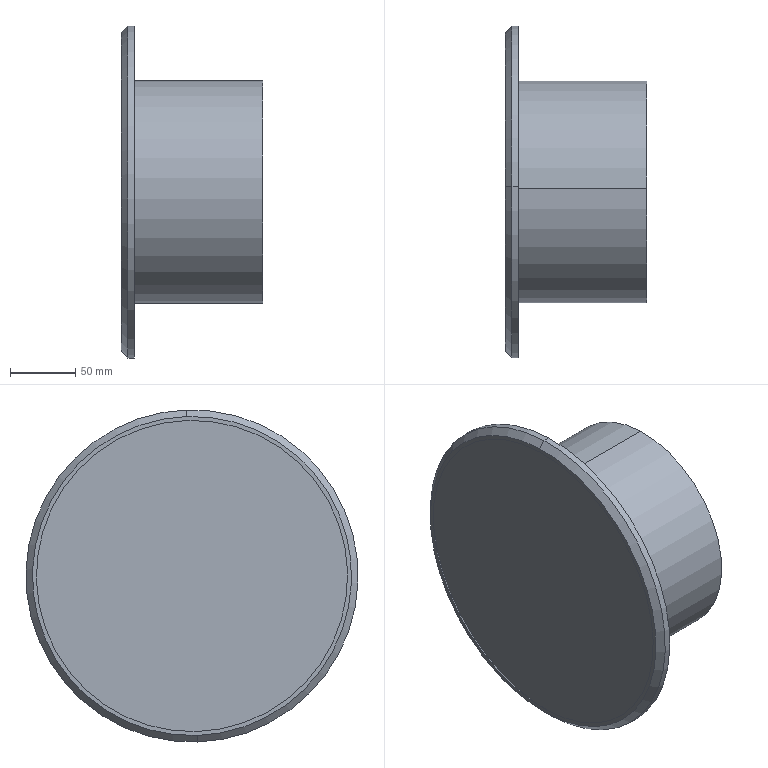Component | SolidWorks | Liner-1 | 1 solid | 15 faces | box 108 x 254 x 254 mm | volume 805465 mm3 | cylinder 6 | plane 5 | cone 4 | commonest cylinder face diameters 254 x2 170 x2 150 x2
build123d program:
from build123d import *

# Parameters (mm, degrees)
CHAMFER2_SIZE = 5


with BuildPart() as part:
    # Sketch1 → Revolve1 (revolve)
    with BuildSketch(Plane.XY, mode=Mode.PRIVATE) as revolve1_sk:
        Polygon((108, 75), (108, 85), (10, 85), (10, 127), (0, 127), (0, 119), (4, 123), (4, 0), (10, 0), (10, 75), align=None)
    revolve(revolve1_sk.sketch.rotate(Axis((0, 0, 0), (1, 0, 0)), 90), axis=Axis((0, 0, 0), (1, 0, 0)))

    # Chamfer2
    chamfer2_edges = [part.edges().sort_by_distance(p)[0] for p in [
        (0, 0, -127),
    ]]
    chamfer(chamfer2_edges, length=CHAMFER2_SIZE)


solid = part.part

# Placed as in the assembly
solid = solid.moved(Location((-257.5, 0, 0), (0, 0, 0)))
STEP:
#1=COLOUR_RGB('',0.7922,0.8196,0.9333);
#2=FILL_AREA_STYLE_COLOUR('',#1);
#3=FILL_AREA_STYLE('',(#2));
#4=SURFACE_STYLE_FILL_AREA(#3);
#5=SURFACE_SIDE_STYLE('',(#4));
#6=SURFACE_STYLE_USAGE(.BOTH.,#5);
#7=PRESENTATION_STYLE_ASSIGNMENT((#6));
#8=CARTESIAN_POINT('',(-10.138,0.1561,4.801));
#9=VERTEX_POINT('',#8);
#10=CARTESIAN_POINT('',(-10.138,-0.1561,-4.801));
#11=VERTEX_POINT('',#10);
#12=CARTESIAN_POINT('',(-10.138,-0.,0.));
#13=DIRECTION('',(-1.,-0.,0.));
#14=DIRECTION('',(-0.,-0.0325,-0.9995));
#15=AXIS2_PLACEMENT_3D('',#12,#13,#14);
#16=CIRCLE('',#15,4.803);
#17=EDGE_CURVE('',#9,#11,#16,.T.);
#18=ORIENTED_EDGE('',*,*,#17,.F.);
#19=CARTESIAN_POINT('',(-9.941,0.1625,4.997));
#20=VERTEX_POINT('',#19);
#21=CARTESIAN_POINT('',(-10.138,0.1561,4.801));
#22=DIRECTION('',(0.7071,0.02298,0.7067));
#23=VECTOR('',#22,39.37);
#24=LINE('',#21,#23);
#25=EDGE_CURVE('',#9,#20,#24,.T.);
#26=ORIENTED_EDGE('',*,*,#25,.T.);
#27=CARTESIAN_POINT('',(-9.941,-0.1625,-4.997));
#28=VERTEX_POINT('',#27);
#29=CARTESIAN_POINT('',(-9.941,-0.,0.));
#30=DIRECTION('',(1.,0.,-0.));
#31=DIRECTION('',(-0.,-0.0325,-0.9995));
#32=AXIS2_PLACEMENT_3D('',#29,#30,#31);
#33=CIRCLE('',#32,5.);
#34=EDGE_CURVE('',#28,#20,#33,.T.);
#35=ORIENTED_EDGE('',*,*,#34,.F.);
#36=CARTESIAN_POINT('',(-10.138,-0.1561,-4.801));
#37=DIRECTION('',(0.7071,-0.02298,-0.7067));
#38=VECTOR('',#37,39.37);
#39=LINE('',#36,#38);
#40=EDGE_CURVE('',#11,#28,#39,.T.);
#41=ORIENTED_EDGE('',*,*,#40,.F.);
#42=EDGE_LOOP('',(#18,#26,#35,#41));
#43=FACE_OUTER_BOUND('',#42,.T.);
#44=CARTESIAN_POINT('',(-10.138,-0.,0.));
#45=DIRECTION('',(1.,0.,-0.));
#46=DIRECTION('',(-0.,-0.0325,-0.9995));
#47=AXIS2_PLACEMENT_3D('',#44,#45,#46);
#48=CONICAL_SURFACE('',#47,4.803,0.7854);
#49=ADVANCED_FACE('',(#43),#48,.T.);
#50=CARTESIAN_POINT('',(-10.138,-0.1523,-4.683));
#51=VERTEX_POINT('',#50);
#52=CARTESIAN_POINT('',(-10.138,0.1523,4.683));
#53=VERTEX_POINT('',#52);
#54=CARTESIAN_POINT('',(-10.138,-0.,0.));
#55=DIRECTION('',(-1.,-0.,0.));
#56=DIRECTION('',(0.,0.0325,0.9995));
#57=AXIS2_PLACEMENT_3D('',#54,#55,#56);
#58=CIRCLE('',#57,4.685);
#59=EDGE_CURVE('',#51,#53,#58,.T.);
#60=ORIENTED_EDGE('',*,*,#59,.T.);
#61=CARTESIAN_POINT('',(-9.98,0.1574,4.84));
#62=VERTEX_POINT('',#61);
#63=CARTESIAN_POINT('',(-10.138,0.1523,4.683));
#64=DIRECTION('',(0.7071,0.02298,0.7067));
#65=VECTOR('',#64,39.37);
#66=LINE('',#63,#65);
#67=EDGE_CURVE('',#53,#62,#66,.T.);
#68=ORIENTED_EDGE('',*,*,#67,.T.);
#69=CARTESIAN_POINT('',(-9.98,-0.1574,-4.84));
#70=VERTEX_POINT('',#69);
#71=CARTESIAN_POINT('',(-9.98,-0.,0.));
#72=DIRECTION('',(-1.,-0.,0.));
#73=DIRECTION('',(0.,0.0325,0.9995));
#74=AXIS2_PLACEMENT_3D('',#71,#72,#73);
#75=CIRCLE('',#74,4.843);
#76=EDGE_CURVE('',#70,#62,#75,.T.);
#77=ORIENTED_EDGE('',*,*,#76,.F.);
#78=CARTESIAN_POINT('',(-10.138,-0.1523,-4.683));
#79=DIRECTION('',(0.7071,-0.02298,-0.7067));
#80=VECTOR('',#79,39.37);
#81=LINE('',#78,#80);
#82=EDGE_CURVE('',#51,#70,#81,.T.);
#83=ORIENTED_EDGE('',*,*,#82,.F.);
#84=EDGE_LOOP('',(#60,#68,#77,#83));
#85=FACE_OUTER_BOUND('',#84,.T.);
#86=CARTESIAN_POINT('',(-10.138,-0.,0.));
#87=DIRECTION('',(1.,0.,-0.));
#88=DIRECTION('',(-0.,-0.0325,-0.9995));
#89=AXIS2_PLACEMENT_3D('',#86,#87,#88);
#90=CONICAL_SURFACE('',#89,4.685,0.7854);
#91=ADVANCED_FACE('',(#85),#90,.F.);
#92=CARTESIAN_POINT('',(-9.744,0.1625,4.997));
#93=VERTEX_POINT('',#92);
#94=CARTESIAN_POINT('',(-9.744,-0.1625,-4.997));
#95=VERTEX_POINT('',#94);
#96=CARTESIAN_POINT('',(-9.744,-0.,0.));
#97=DIRECTION('',(-1.,-0.,0.));
#98=DIRECTION('',(0.,0.0325,0.9995));
#99=AXIS2_PLACEMENT_3D('',#96,#97,#98);
#100=CIRCLE('',#99,5.);
#101=EDGE_CURVE('',#93,#95,#100,.T.);
#102=ORIENTED_EDGE('',*,*,#101,.T.);
#103=CARTESIAN_POINT('',(-10.138,-0.1625,-4.997));
#104=DIRECTION('',(-1.,-0.,0.));
#105=VECTOR('',#104,39.37);
#106=LINE('',#103,#105);
#107=EDGE_CURVE('',#95,#28,#106,.T.);
#108=ORIENTED_EDGE('',*,*,#107,.T.);
#109=ORIENTED_EDGE('',*,*,#34,.T.);
#110=CARTESIAN_POINT('',(-10.138,0.1625,4.997));
#111=DIRECTION('',(-1.,-0.,0.));
#112=VECTOR('',#111,39.37);
#113=LINE('',#110,#112);
#114=EDGE_CURVE('',#93,#20,#113,.T.);
#115=ORIENTED_EDGE('',*,*,#114,.F.);
#116=EDGE_LOOP('',(#102,#108,#109,#115));
#117=FACE_OUTER_BOUND('',#116,.T.);
#118=CARTESIAN_POINT('',(-10.138,-0.,0.));
#119=DIRECTION('',(-1.,-0.,0.));
#120=DIRECTION('',(0.,0.0325,0.9995));
#121=AXIS2_PLACEMENT_3D('',#118,#119,#120);
#122=CYLINDRICAL_SURFACE('',#121,5.);
#123=ADVANCED_FACE('',(#117),#122,.T.);
#124=CARTESIAN_POINT('',(-5.886,0.1088,3.345));
#125=VERTEX_POINT('',#124);
#126=CARTESIAN_POINT('',(-5.886,-0.1088,-3.345));
#127=VERTEX_POINT('',#126);
#128=CARTESIAN_POINT('',(-5.886,-0.,0.));
#129=DIRECTION('',(-1.,-0.,0.));
#130=DIRECTION('',(0.,0.0325,0.9995));
#131=AXIS2_PLACEMENT_3D('',#128,#129,#130);
#132=CIRCLE('',#131,3.346);
#133=EDGE_CURVE('',#125,#127,#132,.T.);
#134=ORIENTED_EDGE('',*,*,#133,.T.);
#135=CARTESIAN_POINT('',(-9.744,-0.1088,-3.345));
#136=VERTEX_POINT('',#135);
#137=CARTESIAN_POINT('',(-10.138,-0.1088,-3.345));
#138=DIRECTION('',(-1.,-0.,0.));
#139=VECTOR('',#138,39.37);
#140=LINE('',#137,#139);
#141=EDGE_CURVE('',#127,#136,#140,.T.);
#142=ORIENTED_EDGE('',*,*,#141,.T.);
#143=CARTESIAN_POINT('',(-9.744,0.1088,3.345));
#144=VERTEX_POINT('',#143);
#145=CARTESIAN_POINT('',(-9.744,-0.,0.));
#146=DIRECTION('',(-1.,-0.,0.));
#147=DIRECTION('',(0.,0.0325,0.9995));
#148=AXIS2_PLACEMENT_3D('',#145,#146,#147);
#149=CIRCLE('',#148,3.346);
#150=EDGE_CURVE('',#144,#136,#149,.T.);
#151=ORIENTED_EDGE('',*,*,#150,.F.);
#152=CARTESIAN_POINT('',(-10.138,0.1088,3.345));
#153=DIRECTION('',(-1.,-0.,0.));
#154=VECTOR('',#153,39.37);
#155=LINE('',#152,#154);
#156=EDGE_CURVE('',#125,#144,#155,.T.);
#157=ORIENTED_EDGE('',*,*,#156,.F.);
#158=EDGE_LOOP('',(#134,#142,#151,#157));
#159=FACE_OUTER_BOUND('',#158,.T.);
#160=CARTESIAN_POINT('',(-10.138,-0.,0.));
#161=DIRECTION('',(-1.,-0.,0.));
#162=DIRECTION('',(0.,0.0325,0.9995));
#163=AXIS2_PLACEMENT_3D('',#160,#161,#162);
#164=CYLINDRICAL_SURFACE('',#163,3.346);
#165=ADVANCED_FACE('',(#159),#164,.T.);
#166=CARTESIAN_POINT('',(-5.886,-0.09596,-2.951));
#167=VERTEX_POINT('',#166);
#168=CARTESIAN_POINT('',(-5.886,0.09596,2.951));
#169=VERTEX_POINT('',#168);
#170=CARTESIAN_POINT('',(-5.886,-0.,0.));
#171=DIRECTION('',(-1.,-0.,0.));
#172=DIRECTION('',(0.,0.0325,0.9995));
#173=AXIS2_PLACEMENT_3D('',#170,#171,#172);
#174=CIRCLE('',#173,2.953);
#175=EDGE_CURVE('',#167,#169,#174,.T.);
#176=ORIENTED_EDGE('',*,*,#175,.F.);
#177=CARTESIAN_POINT('',(-9.744,-0.09596,-2.951));
#178=VERTEX_POINT('',#177);
#179=CARTESIAN_POINT('',(-10.138,-0.09596,-2.951));
#180=DIRECTION('',(-1.,-0.,0.));
#181=VECTOR('',#180,39.37);
#182=LINE('',#179,#181);
#183=EDGE_CURVE('',#167,#178,#182,.T.);
#184=ORIENTED_EDGE('',*,*,#183,.T.);
#185=CARTESIAN_POINT('',(-9.744,0.09596,2.951));
#186=VERTEX_POINT('',#185);
#187=CARTESIAN_POINT('',(-9.744,-0.,0.));
#188=DIRECTION('',(-1.,-0.,0.));
#189=DIRECTION('',(0.,0.0325,0.9995));
#190=AXIS2_PLACEMENT_3D('',#187,#188,#189);
#191=CIRCLE('',#190,2.953);
#192=EDGE_CURVE('',#178,#186,#191,.T.);
#193=ORIENTED_EDGE('',*,*,#192,.T.);
#194=CARTESIAN_POINT('',(-10.138,0.09596,2.951));
#195=DIRECTION('',(-1.,-0.,0.));
#196=VECTOR('',#195,39.37);
#197=LINE('',#194,#196);
#198=EDGE_CURVE('',#169,#186,#197,.T.);
#199=ORIENTED_EDGE('',*,*,#198,.F.);
#200=EDGE_LOOP('',(#176,#184,#193,#199));
#201=FACE_OUTER_BOUND('',#200,.T.);
#202=CARTESIAN_POINT('',(-10.138,-0.,0.));
#203=DIRECTION('',(-1.,-0.,0.));
#204=DIRECTION('',(0.,0.0325,0.9995));
#205=AXIS2_PLACEMENT_3D('',#202,#203,#204);
#206=CYLINDRICAL_SURFACE('',#205,2.953);
#207=ADVANCED_FACE('',(#201),#206,.F.);
#208=ORIENTED_EDGE('',*,*,#183,.F.);
#209=CARTESIAN_POINT('',(-5.886,-0.,0.));
#210=DIRECTION('',(-1.,-0.,0.));
#211=DIRECTION('',(0.,0.0325,0.9995));
#212=AXIS2_PLACEMENT_3D('',#209,#210,#211);
#213=CIRCLE('',#212,2.953);
#214=EDGE_CURVE('',#169,#167,#213,.T.);
#215=ORIENTED_EDGE('',*,*,#214,.F.);
#216=ORIENTED_EDGE('',*,*,#198,.T.);
#217=CARTESIAN_POINT('',(-9.744,-0.,0.));
#218=DIRECTION('',(-1.,-0.,0.));
#219=DIRECTION('',(0.,0.0325,0.9995));
#220=AXIS2_PLACEMENT_3D('',#217,#218,#219);
#221=CIRCLE('',#220,2.953);
#222=EDGE_CURVE('',#186,#178,#221,.T.);
#223=ORIENTED_EDGE('',*,*,#222,.T.);
#224=EDGE_LOOP('',(#208,#215,#216,#223));
#225=FACE_OUTER_BOUND('',#224,.T.);
#226=CARTESIAN_POINT('',(-10.138,-0.,0.));
#227=DIRECTION('',(-1.,-0.,0.));
#228=DIRECTION('',(0.,0.0325,0.9995));
#229=AXIS2_PLACEMENT_3D('',#226,#227,#228);
#230=CYLINDRICAL_SURFACE('',#229,2.953);
#231=ADVANCED_FACE('',(#225),#230,.F.);
#232=ORIENTED_EDGE('',*,*,#133,.F.);
#233=CARTESIAN_POINT('',(-5.886,-0.,0.));
#234=DIRECTION('',(-1.,-0.,0.));
#235=DIRECTION('',(0.,0.0325,0.9995));
#236=AXIS2_PLACEMENT_3D('',#233,#234,#235);
#237=CIRCLE('',#236,3.346);
#238=EDGE_CURVE('',#127,#125,#237,.T.);
#239=ORIENTED_EDGE('',*,*,#238,.F.);
#240=EDGE_LOOP('',(#232,#239));
#241=FACE_OUTER_BOUND('',#240,.T.);
#242=ORIENTED_EDGE('',*,*,#214,.T.);
#243=ORIENTED_EDGE('',*,*,#175,.T.);
#244=EDGE_LOOP('',(#242,#243));
#245=FACE_BOUND('',#244,.T.);
#246=CARTESIAN_POINT('',(-5.886,2.951,-0.09596));
#247=DIRECTION('',(-1.,-0.,0.));
#248=DIRECTION('',(0.,0.0325,0.9995));
#249=AXIS2_PLACEMENT_3D('',#246,#247,#248);
#250=PLANE('',#249);
#251=ADVANCED_FACE('',(#241,#245),#250,.F.);
#252=ORIENTED_EDGE('',*,*,#141,.F.);
#253=ORIENTED_EDGE('',*,*,#238,.T.);
#254=ORIENTED_EDGE('',*,*,#156,.T.);
#255=CARTESIAN_POINT('',(-9.744,-0.,0.));
#256=DIRECTION('',(-1.,-0.,0.));
#257=DIRECTION('',(0.,0.0325,0.9995));
#258=AXIS2_PLACEMENT_3D('',#255,#256,#257);
#259=CIRCLE('',#258,3.346);
#260=EDGE_CURVE('',#136,#144,#259,.T.);
#261=ORIENTED_EDGE('',*,*,#260,.F.);
#262=EDGE_LOOP('',(#252,#253,#254,#261));
#263=FACE_OUTER_BOUND('',#262,.T.);
#264=CARTESIAN_POINT('',(-10.138,-0.,0.));
#265=DIRECTION('',(-1.,-0.,0.));
#266=DIRECTION('',(0.,0.0325,0.9995));
#267=AXIS2_PLACEMENT_3D('',#264,#265,#266);
#268=CYLINDRICAL_SURFACE('',#267,3.346);
#269=ADVANCED_FACE('',(#263),#268,.T.);
#270=ORIENTED_EDGE('',*,*,#101,.F.);
#271=CARTESIAN_POINT('',(-9.744,-0.,0.));
#272=DIRECTION('',(-1.,-0.,0.));
#273=DIRECTION('',(0.,0.0325,0.9995));
#274=AXIS2_PLACEMENT_3D('',#271,#272,#273);
#275=CIRCLE('',#274,5.);
#276=EDGE_CURVE('',#95,#93,#275,.T.);
#277=ORIENTED_EDGE('',*,*,#276,.F.);
#278=EDGE_LOOP('',(#270,#277));
#279=FACE_OUTER_BOUND('',#278,.T.);
#280=ORIENTED_EDGE('',*,*,#150,.T.);
#281=ORIENTED_EDGE('',*,*,#260,.T.);
#282=EDGE_LOOP('',(#280,#281));
#283=FACE_BOUND('',#282,.T.);
#284=CARTESIAN_POINT('',(-9.744,3.345,-0.1088));
#285=DIRECTION('',(-1.,-0.,0.));
#286=DIRECTION('',(0.,0.0325,0.9995));
#287=AXIS2_PLACEMENT_3D('',#284,#285,#286);
#288=PLANE('',#287);
#289=ADVANCED_FACE('',(#279,#283),#288,.F.);
#290=ORIENTED_EDGE('',*,*,#107,.F.);
#291=ORIENTED_EDGE('',*,*,#276,.T.);
#292=ORIENTED_EDGE('',*,*,#114,.T.);
#293=CARTESIAN_POINT('',(-9.941,-0.,0.));
#294=DIRECTION('',(1.,0.,-0.));
#295=DIRECTION('',(-0.,-0.0325,-0.9995));
#296=AXIS2_PLACEMENT_3D('',#293,#294,#295);
#297=CIRCLE('',#296,5.);
#298=EDGE_CURVE('',#20,#28,#297,.T.);
#299=ORIENTED_EDGE('',*,*,#298,.T.);
#300=EDGE_LOOP('',(#290,#291,#292,#299));
#301=FACE_OUTER_BOUND('',#300,.T.);
#302=CARTESIAN_POINT('',(-10.138,-0.,0.));
#303=DIRECTION('',(-1.,-0.,0.));
#304=DIRECTION('',(0.,0.0325,0.9995));
#305=AXIS2_PLACEMENT_3D('',#302,#303,#304);
#306=CYLINDRICAL_SURFACE('',#305,5.);
#307=ADVANCED_FACE('',(#301),#306,.T.);
#308=CARTESIAN_POINT('',(-10.138,-0.,0.));
#309=DIRECTION('',(-1.,-0.,0.));
#310=DIRECTION('',(-0.,-0.0325,-0.9995));
#311=AXIS2_PLACEMENT_3D('',#308,#309,#310);
#312=CIRCLE('',#311,4.803);
#313=EDGE_CURVE('',#11,#9,#312,.T.);
#314=ORIENTED_EDGE('',*,*,#313,.T.);
#315=ORIENTED_EDGE('',*,*,#17,.T.);
#316=EDGE_LOOP('',(#314,#315));
#317=FACE_OUTER_BOUND('',#316,.T.);
#318=ORIENTED_EDGE('',*,*,#59,.F.);
#319=CARTESIAN_POINT('',(-10.138,-0.,0.));
#320=DIRECTION('',(-1.,-0.,0.));
#321=DIRECTION('',(0.,0.0325,0.9995));
#322=AXIS2_PLACEMENT_3D('',#319,#320,#321);
#323=CIRCLE('',#322,4.685);
#324=EDGE_CURVE('',#53,#51,#323,.T.);
#325=ORIENTED_EDGE('',*,*,#324,.F.);
#326=EDGE_LOOP('',(#318,#325));
#327=FACE_BOUND('',#326,.T.);
#328=CARTESIAN_POINT('',(-10.138,4.997,-0.1625));
#329=DIRECTION('',(1.,0.,-0.));
#330=DIRECTION('',(-0.,-0.0325,-0.9995));
#331=AXIS2_PLACEMENT_3D('',#328,#329,#330);
#332=PLANE('',#331);
#333=ADVANCED_FACE('',(#317,#327),#332,.F.);
#334=ORIENTED_EDGE('',*,*,#67,.F.);
#335=ORIENTED_EDGE('',*,*,#324,.T.);
#336=ORIENTED_EDGE('',*,*,#82,.T.);
#337=CARTESIAN_POINT('',(-9.98,-0.,0.));
#338=DIRECTION('',(-1.,-0.,0.));
#339=DIRECTION('',(0.,0.0325,0.9995));
#340=AXIS2_PLACEMENT_3D('',#337,#338,#339);
#341=CIRCLE('',#340,4.843);
#342=EDGE_CURVE('',#62,#70,#341,.T.);
#343=ORIENTED_EDGE('',*,*,#342,.F.);
#344=EDGE_LOOP('',(#334,#335,#336,#343));
#345=FACE_OUTER_BOUND('',#344,.T.);
#346=CARTESIAN_POINT('',(-10.138,-0.,0.));
#347=DIRECTION('',(1.,0.,-0.));
#348=DIRECTION('',(-0.,-0.0325,-0.9995));
#349=AXIS2_PLACEMENT_3D('',#346,#347,#348);
#350=CONICAL_SURFACE('',#349,4.685,0.7854);
#351=ADVANCED_FACE('',(#345),#350,.F.);
#352=ORIENTED_EDGE('',*,*,#76,.T.);
#353=ORIENTED_EDGE('',*,*,#342,.T.);
#354=EDGE_LOOP('',(#352,#353));
#355=FACE_OUTER_BOUND('',#354,.T.);
#356=CARTESIAN_POINT('',(-9.98,4.84,-0.1574));
#357=DIRECTION('',(1.,0.,-0.));
#358=DIRECTION('',(-0.,-0.0325,-0.9995));
#359=AXIS2_PLACEMENT_3D('',#356,#357,#358);
#360=PLANE('',#359);
#361=ADVANCED_FACE('',(#355),#360,.F.);
#362=ORIENTED_EDGE('',*,*,#222,.F.);
#363=ORIENTED_EDGE('',*,*,#192,.F.);
#364=EDGE_LOOP('',(#362,#363));
#365=FACE_OUTER_BOUND('',#364,.T.);
#366=CARTESIAN_POINT('',(-9.744,2.951,-0.09596));
#367=DIRECTION('',(-1.,-0.,0.));
#368=DIRECTION('',(0.,0.0325,0.9995));
#369=AXIS2_PLACEMENT_3D('',#366,#367,#368);
#370=PLANE('',#369);
#371=ADVANCED_FACE('',(#365),#370,.F.);
#372=ORIENTED_EDGE('',*,*,#25,.F.);
#373=ORIENTED_EDGE('',*,*,#313,.F.);
#374=ORIENTED_EDGE('',*,*,#40,.T.);
#375=ORIENTED_EDGE('',*,*,#298,.F.);
#376=EDGE_LOOP('',(#372,#373,#374,#375));
#377=FACE_OUTER_BOUND('',#376,.T.);
#378=CARTESIAN_POINT('',(-10.138,-0.,0.));
#379=DIRECTION('',(1.,0.,-0.));
#380=DIRECTION('',(-0.,-0.0325,-0.9995));
#381=AXIS2_PLACEMENT_3D('',#378,#379,#380);
#382=CONICAL_SURFACE('',#381,4.803,0.7854);
#383=ADVANCED_FACE('',(#377),#382,.T.);
#384=CLOSED_SHELL('',(#49,#91,#123,#165,#207,#231,#251,#269,#289,#307,#333,#351,#361,#371,#383));
#385=MANIFOLD_SOLID_BREP('',#384);
#386=STYLED_ITEM('',(#7),#385);
#387=(LENGTH_UNIT()NAMED_UNIT(*)SI_UNIT($,.METRE.));
#388=LENGTH_MEASURE_WITH_UNIT(LENGTH_MEASURE(0.0254),#387);
#389=DIMENSIONAL_EXPONENTS(1.,0.,0.,0.,0.,0.,0.);
#390=(CONVERSION_BASED_UNIT('',#388)LENGTH_UNIT()NAMED_UNIT(#389));
#391=UNCERTAINTY_MEASURE_WITH_UNIT(LENGTH_MEASURE(0.00001),#390,'','');
#392=(NAMED_UNIT(*)PLANE_ANGLE_UNIT()SI_UNIT($,.RADIAN.));
#393=(NAMED_UNIT(*)SI_UNIT($,.STERADIAN.)SOLID_ANGLE_UNIT());
#394=(GEOMETRIC_REPRESENTATION_CONTEXT(3)GLOBAL_UNCERTAINTY_ASSIGNED_CONTEXT((#391))GLOBAL_UNIT_ASSIGNED_CONTEXT((#390,#392,#393))REPRESENTATION_CONTEXT('',''));
#395=MECHANICAL_DESIGN_GEOMETRIC_PRESENTATION_REPRESENTATION('',(#386),#394);
#396=PRESENTATION_LAYER_ASSIGNMENT('','',(#386));
#397=CARTESIAN_POINT('',(0.,0.,0.));
#398=DIRECTION('',(0.,0.,1.));
#399=DIRECTION('',(1.,0.,0.));
#400=AXIS2_PLACEMENT_3D('',#397,#398,#399);
#401=(LENGTH_UNIT()NAMED_UNIT(*)SI_UNIT($,.METRE.));
#402=LENGTH_MEASURE_WITH_UNIT(LENGTH_MEASURE(0.0254),#401);
#403=DIMENSIONAL_EXPONENTS(1.,0.,0.,0.,0.,0.,0.);
#404=(CONVERSION_BASED_UNIT('',#402)LENGTH_UNIT()NAMED_UNIT(#403));
#405=UNCERTAINTY_MEASURE_WITH_UNIT(LENGTH_MEASURE(0.00001),#404,'','');
#406=(NAMED_UNIT(*)PLANE_ANGLE_UNIT()SI_UNIT($,.RADIAN.));
#407=(NAMED_UNIT(*)SI_UNIT($,.STERADIAN.)SOLID_ANGLE_UNIT());
#408=(GEOMETRIC_REPRESENTATION_CONTEXT(3)GLOBAL_UNCERTAINTY_ASSIGNED_CONTEXT((#405))GLOBAL_UNIT_ASSIGNED_CONTEXT((#404,#406,#407))REPRESENTATION_CONTEXT('',''));
#409=ADVANCED_BREP_SHAPE_REPRESENTATION('',(#385,#400),#408);